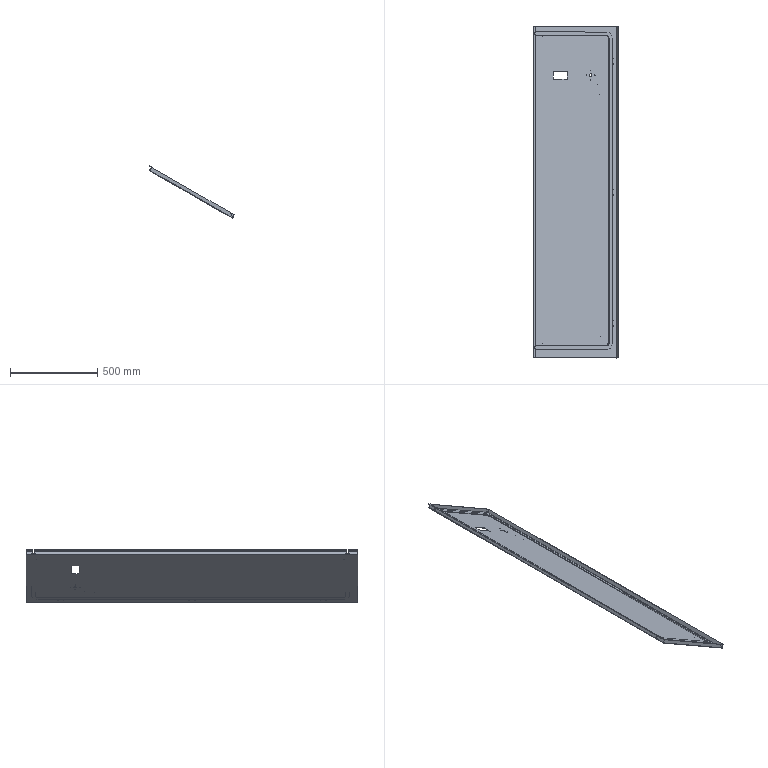Component | SolidWorks | FrontDoorFlangeWelding-2_FrontDoorFlange-1 | 1 solid | 149 faces | volume 2024333 mm3 | plane 87 | cylinder 60 | spline 2 | commonest cylinder face diameters 0.5 x26 3.2 x9 0.2 x9 5.2 x8 17 x2 10 x2 29.934 x2 69.934 x2